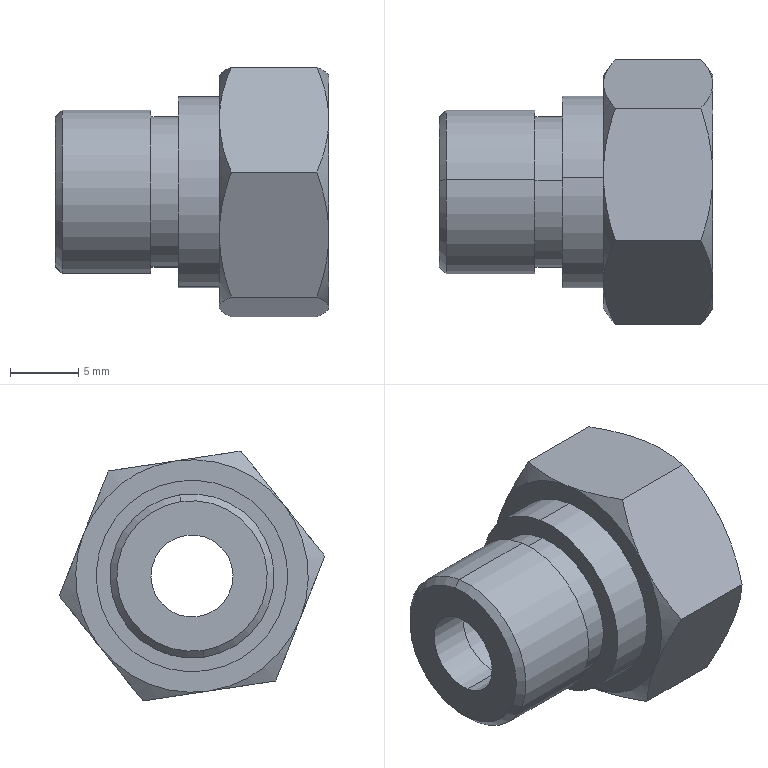Component | SolidWorks | STB-08-000-3-1_STB-08-024-1 | 1 solid | 39 faces | volume 2376 mm3 | cone 14 | plane 13 | cylinder 12 | commonest cylinder face diameters 10 x2 12 x2 11 x2 14 x2 6 x2 8 x2